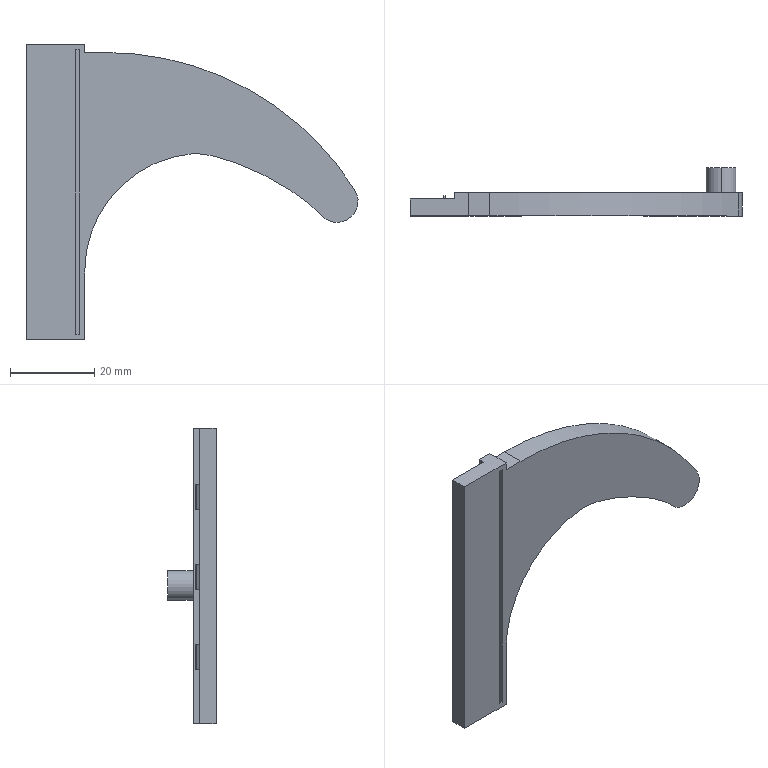Component | SolidWorks | ReversingArmBracket-1 | 4 solids | 94 faces | box 79.04 x 11.5 x 70.4 mm | volume 11280 mm3 | plane 77 | cylinder 16 | spline 1 | commonest cylinder face diameters 140 x6 136 x3 7 x2 10.189 x2 10 x2 56 x1
build123d program:
from build123d import *

# Parameters (mm, degrees)
BOSS_EXTRUDE1_DEPTH      = 2
BOSS_EXTRUDE1_DEPTH_BACK = 2
SKETCH1_W                = 70.4
SKETCH1_H                = 10.5
BOSS_EXTRUDE2_DEPTH      = 3.5
BOSS_EXTRUDE2_DEPTH_BACK = 3
SKETCH2_W                = 70.4
SKETCH2_H                = 3.5
SKETCH2_W_2              = 67.8
SKETCH2_H_2              = 0.9
BOSS_EXTRUDE3_DEPTH      = 1
BOSS_EXTRUDE3_DEPTH_BACK = 1
SKETCH3_W                = 67.8
SKETCH3_H                = 0.9
BOSS_EXTRUDE4_DEPTH      = 3.5
BOSS_EXTRUDE4_DEPTH_BACK = 2
CUT_EXTRUDE1_DEPTH       = 1.5
SKETCH6_R                = 3.5
BOSS_EXTRUDE5_DEPTH      = 6
SKETCH8_W                = 1
SKETCH8_H                = 3.5
CUT_EXTRUDE2_DEPTH       = 75
BOSS_EXTRUDE6_DEPTH      = 70.4
SKETCH10_W               = 16.322
SKETCH10_H               = 3.832
SKETCH10_W_2             = 13
SKETCH10_H_2             = 4.652
SKETCH10_W_3             = 14.7
SKETCH10_H_3             = 6.727
CUT_EXTRUDE3_DEPTH       = 19.4
CUT_EXTRUDE4_DEPTH       = 0.5


with BuildPart() as part:
    # Sketch1 → Boss-Extrude1 (new, two sides: drawn at the far end of the back side and taken through both)
    with BuildSketch(Plane.XY.offset(-BOSS_EXTRUDE1_DEPTH_BACK)):
        with Locations((35.2, 5.25)):
            Rectangle(SKETCH1_W, SKETCH1_H)
    extrude(amount=BOSS_EXTRUDE1_DEPTH + BOSS_EXTRUDE1_DEPTH_BACK)

    # Sketch2 → Boss-Extrude2 (add, two sides: drawn at the far end of the back side and taken through both)
    with BuildSketch(Plane.XY.offset(-BOSS_EXTRUDE2_DEPTH_BACK)):
        with Locations((35.2, 12.25)):
            Rectangle(SKETCH2_W, SKETCH2_H)
        with Locations((35.2, 12.25)):
            Rectangle(SKETCH2_W_2, SKETCH2_H_2, mode=Mode.SUBTRACT)
    extrude(amount=BOSS_EXTRUDE2_DEPTH + BOSS_EXTRUDE2_DEPTH_BACK)

    # Sketch3 → Boss-Extrude3 (add, two sides: drawn at the far end of the back side and taken through both)
    with BuildSketch(Plane.XY.offset(-BOSS_EXTRUDE3_DEPTH_BACK)):
        with Locations((35.2, 12.25)):
            Rectangle(SKETCH3_W, SKETCH3_H)
    extrude(amount=BOSS_EXTRUDE3_DEPTH + BOSS_EXTRUDE3_DEPTH_BACK)

    # Sketch4 → Boss-Extrude4 (add, two sides: drawn at the far end of the back side and taken through both)
    with BuildSketch(Plane.XY.offset(-BOSS_EXTRUDE4_DEPTH_BACK)):
        with BuildLine():
            ThreePointArc((44.27, 39.304), (35.222, 21.27), (16.4, 14))
            Line((16.4, 14), (68.4, 14))
            Line((68.4, 14), (68.4, 19))
            ThreePointArc((68.4, 19), (59.663, 52.865), (35.633, 78.276))
            ThreePointArc((35.633, 78.276), (28.986, 77.058), (29.625, 70.33))
            add(Edge.make_bspline(
                [(29.625, 70.33), (36.749, 63.902), (45.001, 46.865), (44.27, 39.304)],
                knots=[0, 0, 0, 0, 1, 1, 1, 1], degree=3))
        make_face()
    extrude(amount=BOSS_EXTRUDE4_DEPTH + BOSS_EXTRUDE4_DEPTH_BACK)

    # Sketch5 → Cut-Extrude1 (cut)
    with BuildSketch(Plane.XY.offset(3.5)):
        with BuildLine():
            Line((66.4, 19), (51.4, 19))
            ThreePointArc((51.4, 19), (51.474, 21.559), (51.455, 24.118))
            Line((51.455, 24.118), (64.531, 34.835))
            ThreePointArc((64.531, 34.835), (65.931, 26.972), (66.4, 19))
        make_face()
        with BuildLine():
            Line((41.983, 71.197), (39.395, 61.62))
            ThreePointArc((39.395, 61.62), (36.639, 65.402), (33.636, 68.991))
            ThreePointArc((33.636, 68.991), (36.866, 70.755), (38.065, 74.233))
            ThreePointArc((38.065, 74.233), (40.051, 72.751), (41.983, 71.197))
        make_face()
        with BuildLine():
            Line((43.663, 69.747), (40.86, 59.371))
            ThreePointArc((40.86, 59.371), (44.201, 53.383), (46.941, 47.097))
            Line((46.941, 47.097), (63.683, 38.031))
            ThreePointArc((63.683, 38.031), (55.903, 55.297), (43.663, 69.747))
        make_face()
        with BuildLine():
            Line((63.307, 35.96), (51.371, 26.177))
            ThreePointArc((51.371, 26.177), (50.253, 35.343), (47.939, 44.282))
            Line((47.939, 44.282), (63.307, 35.96))
        make_face()
    extrude(amount=-CUT_EXTRUDE1_DEPTH, mode=Mode.SUBTRACT)

    # Sketch6 → Boss-Extrude5 (add)
    with BuildSketch(Plane.XY.offset(3.5)):
        with Locations(Location((32.974, 74.042, 0), (0, 0, 180))):
            Circle(SKETCH6_R)
    extrude(amount=BOSS_EXTRUDE5_DEPTH)

    # Sketch8 → Cut-Extrude2 (cut)
    with BuildSketch(Plane(origin=(70.4, 0, 0), x_dir=(0, 0, -1), z_dir=(1, 0, 0))):
        with Locations((2.5, 12.25)):
            Rectangle(SKETCH8_W, SKETCH8_H)
    extrude(amount=-CUT_EXTRUDE2_DEPTH, mode=Mode.SUBTRACT)

    # Sketch11 → Cut-Extrude4 (cut)
    with BuildSketch(Plane.XY.offset(2)):
        Polygon((13, 8.6), (12.5, 8.6), (12.5, 4.1), (19.5, 4.1), (19.5, 8.6), (19, 8.6), (19, 4.6), (13, 4.6), align=None)
        Polygon((38, 8.6), (38, 4.6), (32, 4.6), (32, 8.6), (31.5, 8.6), (31.5, 4.1), (38.5, 4.1), (38.5, 8.6), align=None)
        Polygon((57, 8.6), (57, 4.6), (51, 4.6), (51, 8.6), (50.5, 8.6), (50.5, 4.1), (57.5, 4.1), (57.5, 8.6), align=None)
    extrude(amount=-CUT_EXTRUDE4_DEPTH, mode=Mode.SUBTRACT)


with BuildPart() as body_2:
    # Sketch9 → Boss-Extrude6 (new body)
    with BuildSketch(Plane(origin=(70.4, 0, 0), x_dir=(0, 0, -1), z_dir=(1, 0, 0))):
        Polygon((-2.8, 8.5), (-2, 8.6), (-2, 7.6), (-2.731, 8.067), align=None)
    extrude(amount=-BOSS_EXTRUDE6_DEPTH)

    # Sketch10 → Cut-Extrude3 (cut)
    with BuildSketch(Plane.XY.offset(2)):
        with Locations((4.839, 7.565)):
            Rectangle(SKETCH10_W, SKETCH10_H)
        with Locations((25.5, 7.155)):
            Rectangle(SKETCH10_W_2, SKETCH10_H_2)
        with Locations((44.5, 7.155)):
            Rectangle(SKETCH10_W_2, SKETCH10_H_2)
        with Locations((64.35, 7.137)):
            Rectangle(SKETCH10_W_3, SKETCH10_H_3)
    extrude(amount=CUT_EXTRUDE3_DEPTH, mode=Mode.SUBTRACT)


with BuildPart() as cut_extrude3_piece_1:
    # of the separate pieces the step leaves, piece 1, a body of its own (cut_extrude3_pieces)
    add(body_2.part.solids().sort_by_distance((38, 8.6, 2))[0])


with BuildPart() as cut_extrude3_piece_2:
    # of the separate pieces the step leaves, piece 2, a body of its own (cut_extrude3_pieces)
    add(body_2.part.solids().sort_by_distance((19, 8.6, 2))[0])


with BuildPart() as cut_extrude3_piece_3:
    # of the separate pieces the step leaves, piece 3, a body of its own (cut_extrude3_pieces)
    add(body_2.part.solids().sort_by_distance((57, 8.6, 2))[0])


solid = Compound([part.part, cut_extrude3_piece_1.part, cut_extrude3_piece_2.part, cut_extrude3_piece_3.part])

# Placed as in the assembly
solid = solid.moved(Location((22.207, 8.747, 1820.664), (-90, 0, -90)))